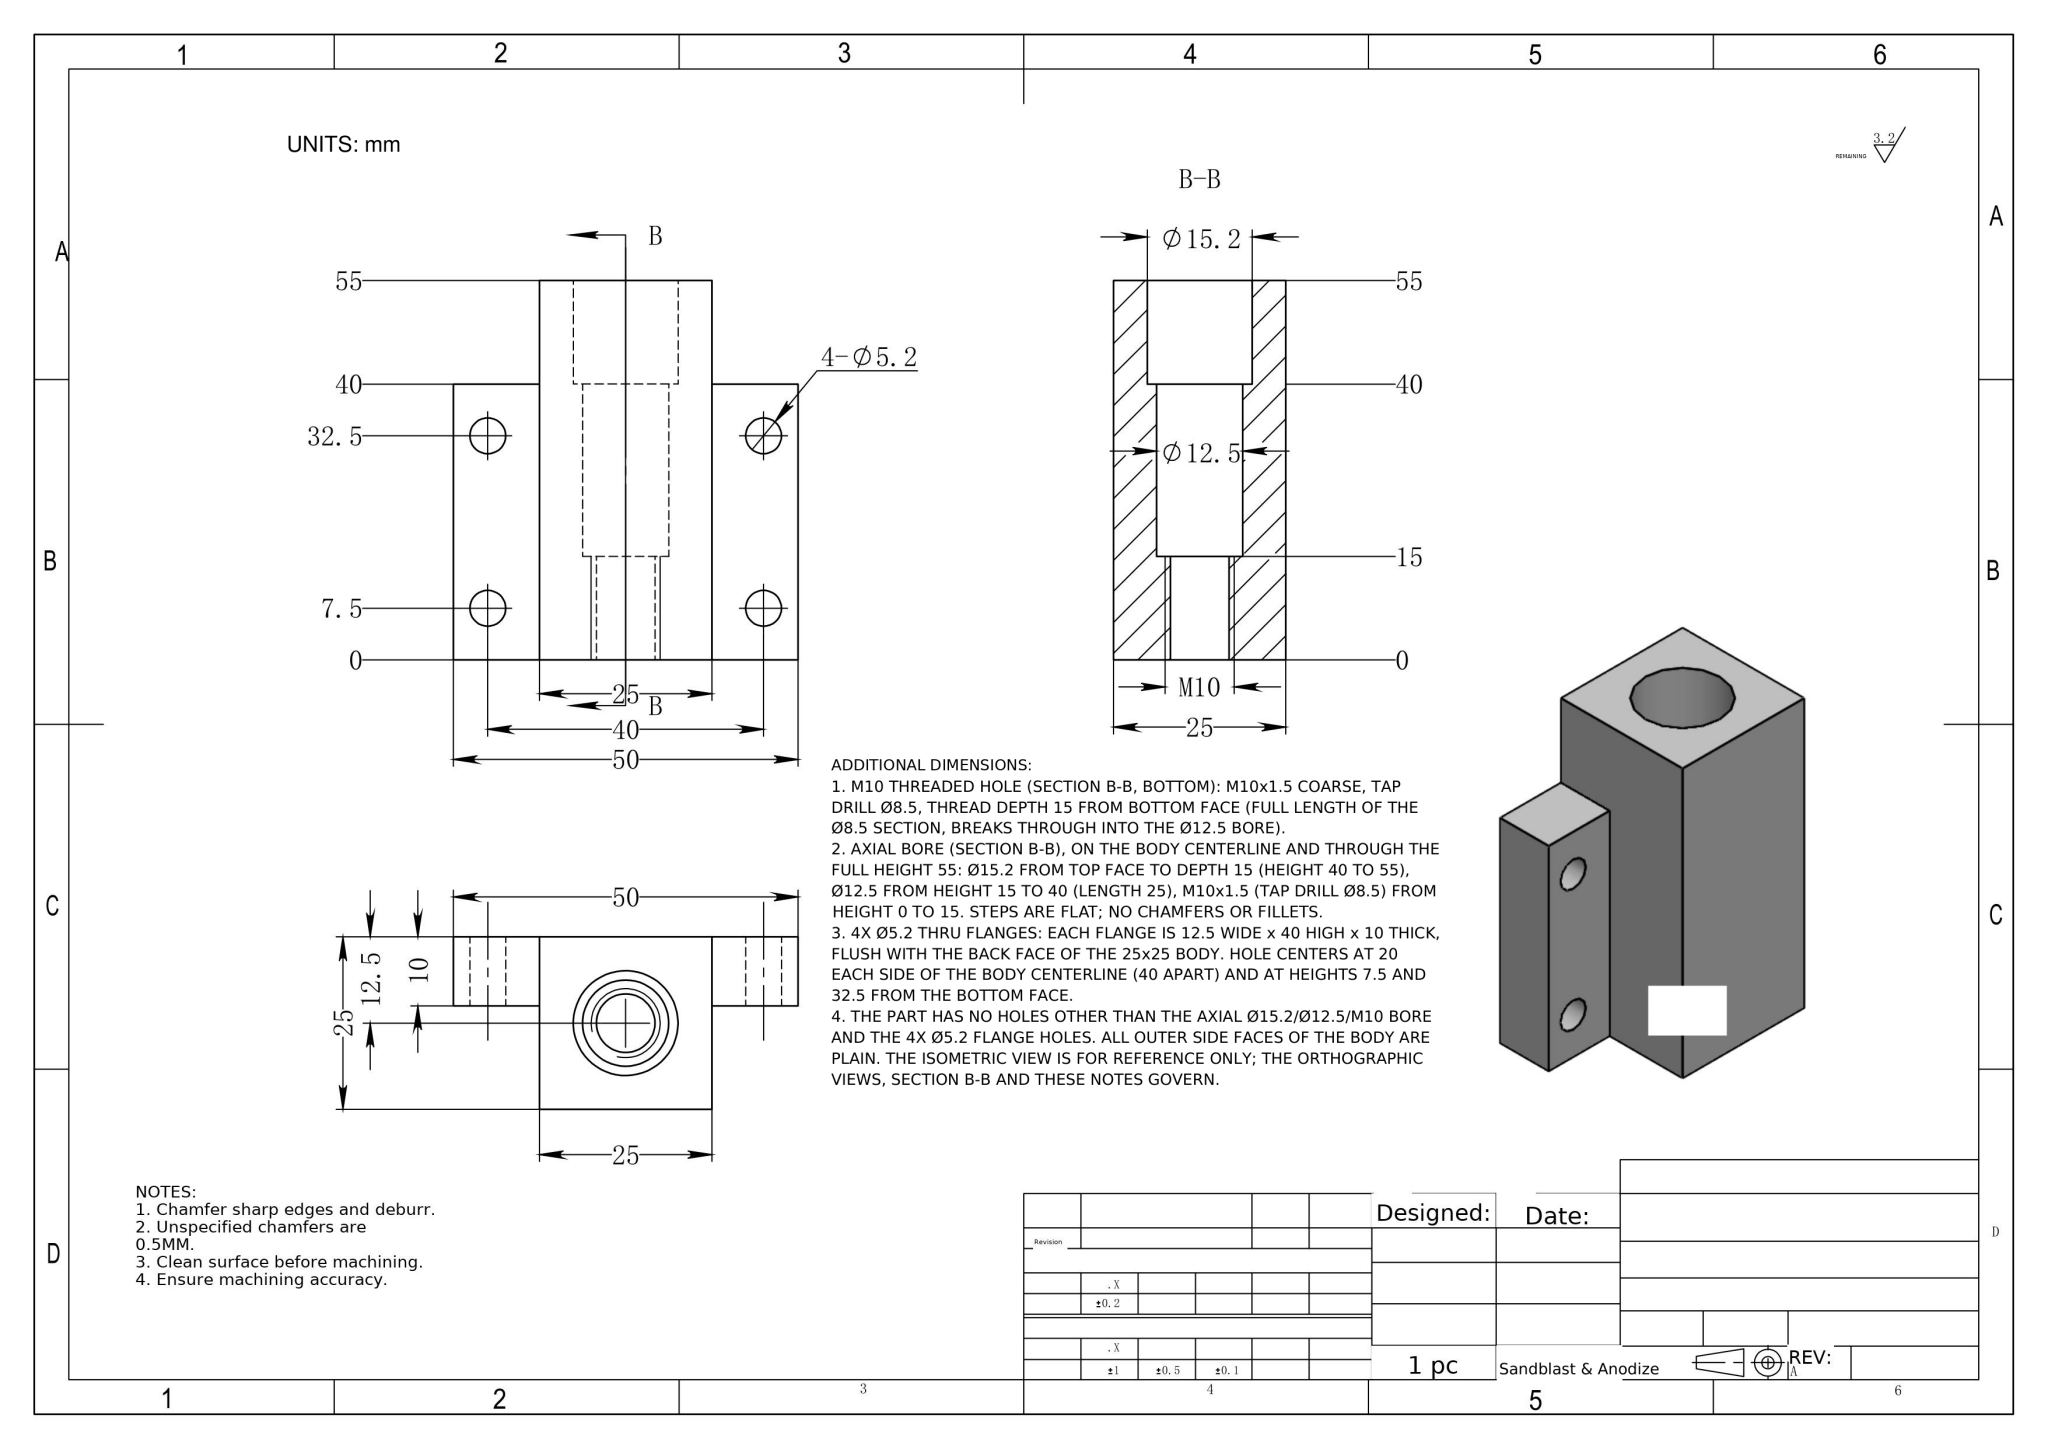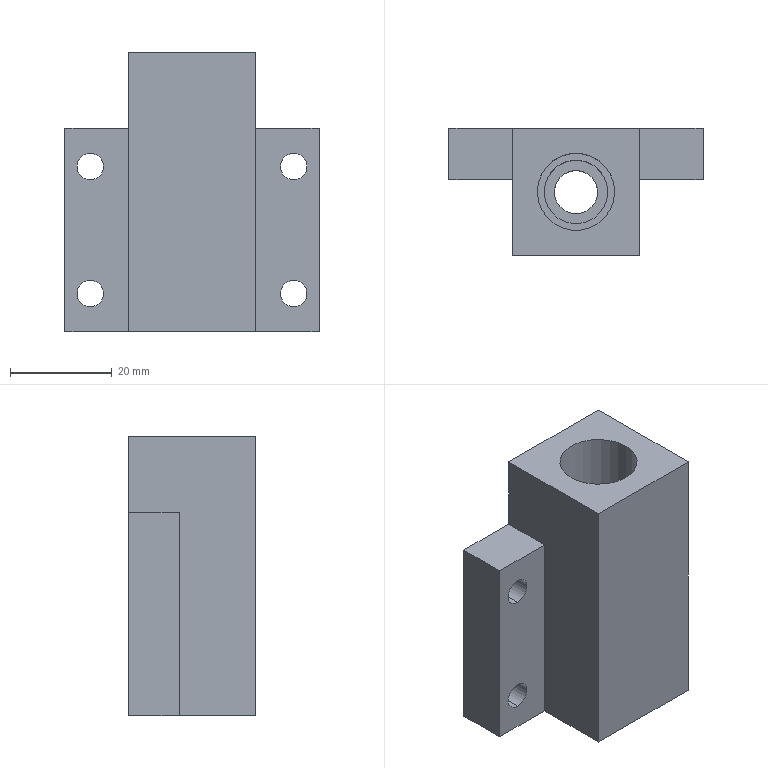Part | NX | mm | 1 solid | 28 faces | box 50 x 25 x 55 mm | volume 36885 mm3 | cylinder 14 | plane 14 | commonest cylinder face diameters 5.2 x8 8.5 x2 12.5 x2 15.2 x2
STEP:
#1=COLOUR_RGB('',1.,1.,1.);
#2=FILL_AREA_STYLE_COLOUR('',#1);
#3=FILL_AREA_STYLE('',(#2));
#4=SURFACE_STYLE_FILL_AREA(#3);
#5=SURFACE_SIDE_STYLE('',(#4));
#6=SURFACE_STYLE_USAGE(.BOTH.,#5);
#7=PRESENTATION_STYLE_ASSIGNMENT((#6));
#8=CARTESIAN_POINT('',(-4.25,0.,15.));
#9=VERTEX_POINT('',#8);
#10=CARTESIAN_POINT('',(4.25,0.,15.));
#11=VERTEX_POINT('',#10);
#12=CARTESIAN_POINT('',(0.,0.,15.));
#13=DIRECTION('',(0.,0.,1.));
#14=DIRECTION('',(1.,0.,0.));
#15=AXIS2_PLACEMENT_3D('',#12,#13,#14);
#16=CIRCLE('',#15,4.25);
#17=EDGE_CURVE('',#9,#11,#16,.T.);
#18=ORIENTED_EDGE('',*,*,#17,.T.);
#19=CARTESIAN_POINT('',(4.25,0.,0.));
#20=VERTEX_POINT('',#19);
#21=CARTESIAN_POINT('',(4.25,0.,0.));
#22=DIRECTION('',(0.,0.,-1.));
#23=VECTOR('',#22,1000.);
#24=LINE('',#21,#23);
#25=EDGE_CURVE('',#11,#20,#24,.T.);
#26=ORIENTED_EDGE('',*,*,#25,.T.);
#27=CARTESIAN_POINT('',(-4.25,0.,0.));
#28=VERTEX_POINT('',#27);
#29=CARTESIAN_POINT('',(0.,0.,0.));
#30=DIRECTION('',(0.,0.,-1.));
#31=DIRECTION('',(-1.,0.,0.));
#32=AXIS2_PLACEMENT_3D('',#29,#30,#31);
#33=CIRCLE('',#32,4.25);
#34=EDGE_CURVE('',#20,#28,#33,.T.);
#35=ORIENTED_EDGE('',*,*,#34,.T.);
#36=CARTESIAN_POINT('',(-4.25,0.,0.));
#37=DIRECTION('',(0.,0.,-1.));
#38=VECTOR('',#37,1000.);
#39=LINE('',#36,#38);
#40=EDGE_CURVE('',#9,#28,#39,.T.);
#41=ORIENTED_EDGE('',*,*,#40,.F.);
#42=EDGE_LOOP('',(#18,#26,#35,#41));
#43=FACE_OUTER_BOUND('',#42,.T.);
#44=CARTESIAN_POINT('',(0.,0.,0.));
#45=DIRECTION('',(0.,0.,-1.));
#46=DIRECTION('',(-1.,0.,0.));
#47=AXIS2_PLACEMENT_3D('',#44,#45,#46);
#48=CYLINDRICAL_SURFACE('',#47,4.25);
#49=ADVANCED_FACE('',(#43),#48,.F.);
#50=CARTESIAN_POINT('',(-6.25,0.,15.));
#51=VERTEX_POINT('',#50);
#52=CARTESIAN_POINT('',(6.25,0.,15.));
#53=VERTEX_POINT('',#52);
#54=CARTESIAN_POINT('',(0.,0.,15.));
#55=DIRECTION('',(0.,0.,1.));
#56=DIRECTION('',(1.,0.,0.));
#57=AXIS2_PLACEMENT_3D('',#54,#55,#56);
#58=CIRCLE('',#57,6.25);
#59=EDGE_CURVE('',#51,#53,#58,.T.);
#60=ORIENTED_EDGE('',*,*,#59,.F.);
#61=CARTESIAN_POINT('',(-6.25,0.,40.));
#62=VERTEX_POINT('',#61);
#63=CARTESIAN_POINT('',(-6.25,0.,15.));
#64=DIRECTION('',(0.,0.,1.));
#65=VECTOR('',#64,1000.);
#66=LINE('',#63,#65);
#67=EDGE_CURVE('',#51,#62,#66,.T.);
#68=ORIENTED_EDGE('',*,*,#67,.T.);
#69=CARTESIAN_POINT('',(6.25,0.,40.));
#70=VERTEX_POINT('',#69);
#71=CARTESIAN_POINT('',(0.,0.,40.));
#72=DIRECTION('',(0.,0.,1.));
#73=DIRECTION('',(1.,0.,0.));
#74=AXIS2_PLACEMENT_3D('',#71,#72,#73);
#75=CIRCLE('',#74,6.25);
#76=EDGE_CURVE('',#62,#70,#75,.T.);
#77=ORIENTED_EDGE('',*,*,#76,.T.);
#78=CARTESIAN_POINT('',(6.25,0.,15.));
#79=DIRECTION('',(0.,0.,1.));
#80=VECTOR('',#79,1000.);
#81=LINE('',#78,#80);
#82=EDGE_CURVE('',#53,#70,#81,.T.);
#83=ORIENTED_EDGE('',*,*,#82,.F.);
#84=EDGE_LOOP('',(#60,#68,#77,#83));
#85=FACE_OUTER_BOUND('',#84,.T.);
#86=CARTESIAN_POINT('',(0.,0.,15.));
#87=DIRECTION('',(0.,0.,1.));
#88=DIRECTION('',(1.,0.,0.));
#89=AXIS2_PLACEMENT_3D('',#86,#87,#88);
#90=CYLINDRICAL_SURFACE('',#89,6.25);
#91=ADVANCED_FACE('',(#85),#90,.F.);
#92=CARTESIAN_POINT('',(-7.6,0.,40.));
#93=VERTEX_POINT('',#92);
#94=CARTESIAN_POINT('',(7.6,0.,40.));
#95=VERTEX_POINT('',#94);
#96=CARTESIAN_POINT('',(0.,0.,40.));
#97=DIRECTION('',(0.,0.,1.));
#98=DIRECTION('',(1.,0.,0.));
#99=AXIS2_PLACEMENT_3D('',#96,#97,#98);
#100=CIRCLE('',#99,7.6);
#101=EDGE_CURVE('',#93,#95,#100,.T.);
#102=ORIENTED_EDGE('',*,*,#101,.F.);
#103=CARTESIAN_POINT('',(-7.6,0.,55.));
#104=VERTEX_POINT('',#103);
#105=CARTESIAN_POINT('',(-7.6,0.,40.));
#106=DIRECTION('',(0.,0.,1.));
#107=VECTOR('',#106,1000.);
#108=LINE('',#105,#107);
#109=EDGE_CURVE('',#93,#104,#108,.T.);
#110=ORIENTED_EDGE('',*,*,#109,.T.);
#111=CARTESIAN_POINT('',(7.6,0.,55.));
#112=VERTEX_POINT('',#111);
#113=CARTESIAN_POINT('',(0.,0.,55.));
#114=DIRECTION('',(0.,0.,1.));
#115=DIRECTION('',(1.,0.,0.));
#116=AXIS2_PLACEMENT_3D('',#113,#114,#115);
#117=CIRCLE('',#116,7.6);
#118=EDGE_CURVE('',#104,#112,#117,.T.);
#119=ORIENTED_EDGE('',*,*,#118,.T.);
#120=CARTESIAN_POINT('',(7.6,0.,40.));
#121=DIRECTION('',(0.,0.,1.));
#122=VECTOR('',#121,1000.);
#123=LINE('',#120,#122);
#124=EDGE_CURVE('',#95,#112,#123,.T.);
#125=ORIENTED_EDGE('',*,*,#124,.F.);
#126=EDGE_LOOP('',(#102,#110,#119,#125));
#127=FACE_OUTER_BOUND('',#126,.T.);
#128=CARTESIAN_POINT('',(0.,0.,40.));
#129=DIRECTION('',(0.,0.,1.));
#130=DIRECTION('',(1.,0.,0.));
#131=AXIS2_PLACEMENT_3D('',#128,#129,#130);
#132=CYLINDRICAL_SURFACE('',#131,7.6);
#133=ADVANCED_FACE('',(#127),#132,.F.);
#134=CARTESIAN_POINT('',(-20.,12.5,35.1));
#135=VERTEX_POINT('',#134);
#136=CARTESIAN_POINT('',(-20.,12.5,29.9));
#137=VERTEX_POINT('',#136);
#138=CARTESIAN_POINT('',(-20.,12.5,32.5));
#139=DIRECTION('',(0.,-1.,0.));
#140=DIRECTION('',(0.,0.,-1.));
#141=AXIS2_PLACEMENT_3D('',#138,#139,#140);
#142=CIRCLE('',#141,2.6);
#143=EDGE_CURVE('',#135,#137,#142,.T.);
#144=ORIENTED_EDGE('',*,*,#143,.F.);
#145=CARTESIAN_POINT('',(-20.,2.5,35.1));
#146=VERTEX_POINT('',#145);
#147=CARTESIAN_POINT('',(-20.,-12.5,35.1));
#148=DIRECTION('',(0.,-1.,0.));
#149=VECTOR('',#148,1000.);
#150=LINE('',#147,#149);
#151=EDGE_CURVE('',#135,#146,#150,.T.);
#152=ORIENTED_EDGE('',*,*,#151,.T.);
#153=CARTESIAN_POINT('',(-20.,2.5,29.9));
#154=VERTEX_POINT('',#153);
#155=CARTESIAN_POINT('',(-20.,2.5,32.5));
#156=DIRECTION('',(0.,1.,0.));
#157=DIRECTION('',(0.,0.,-1.));
#158=AXIS2_PLACEMENT_3D('',#155,#156,#157);
#159=CIRCLE('',#158,2.6);
#160=EDGE_CURVE('',#154,#146,#159,.T.);
#161=ORIENTED_EDGE('',*,*,#160,.F.);
#162=CARTESIAN_POINT('',(-20.,-12.5,29.9));
#163=DIRECTION('',(0.,-1.,0.));
#164=VECTOR('',#163,1000.);
#165=LINE('',#162,#164);
#166=EDGE_CURVE('',#137,#154,#165,.T.);
#167=ORIENTED_EDGE('',*,*,#166,.F.);
#168=EDGE_LOOP('',(#144,#152,#161,#167));
#169=FACE_OUTER_BOUND('',#168,.T.);
#170=CARTESIAN_POINT('',(-20.,-12.5,32.5));
#171=DIRECTION('',(0.,-1.,0.));
#172=DIRECTION('',(0.,0.,-1.));
#173=AXIS2_PLACEMENT_3D('',#170,#171,#172);
#174=CYLINDRICAL_SURFACE('',#173,2.6);
#175=ADVANCED_FACE('',(#169),#174,.F.);
#176=CARTESIAN_POINT('',(-20.,12.5,10.1));
#177=VERTEX_POINT('',#176);
#178=CARTESIAN_POINT('',(-20.,12.5,4.9));
#179=VERTEX_POINT('',#178);
#180=CARTESIAN_POINT('',(-20.,12.5,7.5));
#181=DIRECTION('',(0.,-1.,0.));
#182=DIRECTION('',(0.,0.,-1.));
#183=AXIS2_PLACEMENT_3D('',#180,#181,#182);
#184=CIRCLE('',#183,2.6);
#185=EDGE_CURVE('',#177,#179,#184,.T.);
#186=ORIENTED_EDGE('',*,*,#185,.F.);
#187=CARTESIAN_POINT('',(-20.,2.5,10.1));
#188=VERTEX_POINT('',#187);
#189=CARTESIAN_POINT('',(-20.,-12.5,10.1));
#190=DIRECTION('',(0.,-1.,0.));
#191=VECTOR('',#190,1000.);
#192=LINE('',#189,#191);
#193=EDGE_CURVE('',#177,#188,#192,.T.);
#194=ORIENTED_EDGE('',*,*,#193,.T.);
#195=CARTESIAN_POINT('',(-20.,2.5,4.9));
#196=VERTEX_POINT('',#195);
#197=CARTESIAN_POINT('',(-20.,2.5,7.5));
#198=DIRECTION('',(0.,1.,0.));
#199=DIRECTION('',(0.,0.,-1.));
#200=AXIS2_PLACEMENT_3D('',#197,#198,#199);
#201=CIRCLE('',#200,2.6);
#202=EDGE_CURVE('',#196,#188,#201,.T.);
#203=ORIENTED_EDGE('',*,*,#202,.F.);
#204=CARTESIAN_POINT('',(-20.,-12.5,4.9));
#205=DIRECTION('',(0.,-1.,0.));
#206=VECTOR('',#205,1000.);
#207=LINE('',#204,#206);
#208=EDGE_CURVE('',#179,#196,#207,.T.);
#209=ORIENTED_EDGE('',*,*,#208,.F.);
#210=EDGE_LOOP('',(#186,#194,#203,#209));
#211=FACE_OUTER_BOUND('',#210,.T.);
#212=CARTESIAN_POINT('',(-20.,-12.5,7.5));
#213=DIRECTION('',(0.,-1.,0.));
#214=DIRECTION('',(0.,0.,-1.));
#215=AXIS2_PLACEMENT_3D('',#212,#213,#214);
#216=CYLINDRICAL_SURFACE('',#215,2.6);
#217=ADVANCED_FACE('',(#211),#216,.F.);
#218=CARTESIAN_POINT('',(20.,12.5,35.1));
#219=VERTEX_POINT('',#218);
#220=CARTESIAN_POINT('',(20.,12.5,29.9));
#221=VERTEX_POINT('',#220);
#222=CARTESIAN_POINT('',(20.,12.5,32.5));
#223=DIRECTION('',(0.,-1.,0.));
#224=DIRECTION('',(0.,0.,-1.));
#225=AXIS2_PLACEMENT_3D('',#222,#223,#224);
#226=CIRCLE('',#225,2.6);
#227=EDGE_CURVE('',#219,#221,#226,.T.);
#228=ORIENTED_EDGE('',*,*,#227,.F.);
#229=CARTESIAN_POINT('',(20.,2.5,35.1));
#230=VERTEX_POINT('',#229);
#231=CARTESIAN_POINT('',(20.,-12.5,35.1));
#232=DIRECTION('',(0.,-1.,0.));
#233=VECTOR('',#232,1000.);
#234=LINE('',#231,#233);
#235=EDGE_CURVE('',#219,#230,#234,.T.);
#236=ORIENTED_EDGE('',*,*,#235,.T.);
#237=CARTESIAN_POINT('',(20.,2.5,29.9));
#238=VERTEX_POINT('',#237);
#239=CARTESIAN_POINT('',(20.,2.5,32.5));
#240=DIRECTION('',(0.,1.,0.));
#241=DIRECTION('',(0.,0.,-1.));
#242=AXIS2_PLACEMENT_3D('',#239,#240,#241);
#243=CIRCLE('',#242,2.6);
#244=EDGE_CURVE('',#238,#230,#243,.T.);
#245=ORIENTED_EDGE('',*,*,#244,.F.);
#246=CARTESIAN_POINT('',(20.,-12.5,29.9));
#247=DIRECTION('',(0.,-1.,0.));
#248=VECTOR('',#247,1000.);
#249=LINE('',#246,#248);
#250=EDGE_CURVE('',#221,#238,#249,.T.);
#251=ORIENTED_EDGE('',*,*,#250,.F.);
#252=EDGE_LOOP('',(#228,#236,#245,#251));
#253=FACE_OUTER_BOUND('',#252,.T.);
#254=CARTESIAN_POINT('',(20.,-12.5,32.5));
#255=DIRECTION('',(0.,-1.,0.));
#256=DIRECTION('',(0.,0.,-1.));
#257=AXIS2_PLACEMENT_3D('',#254,#255,#256);
#258=CYLINDRICAL_SURFACE('',#257,2.6);
#259=ADVANCED_FACE('',(#253),#258,.F.);
#260=CARTESIAN_POINT('',(20.,12.5,10.1));
#261=VERTEX_POINT('',#260);
#262=CARTESIAN_POINT('',(20.,12.5,4.9));
#263=VERTEX_POINT('',#262);
#264=CARTESIAN_POINT('',(20.,12.5,7.5));
#265=DIRECTION('',(0.,-1.,0.));
#266=DIRECTION('',(0.,0.,-1.));
#267=AXIS2_PLACEMENT_3D('',#264,#265,#266);
#268=CIRCLE('',#267,2.6);
#269=EDGE_CURVE('',#261,#263,#268,.T.);
#270=ORIENTED_EDGE('',*,*,#269,.F.);
#271=CARTESIAN_POINT('',(20.,2.5,10.1));
#272=VERTEX_POINT('',#271);
#273=CARTESIAN_POINT('',(20.,-12.5,10.1));
#274=DIRECTION('',(0.,-1.,0.));
#275=VECTOR('',#274,1000.);
#276=LINE('',#273,#275);
#277=EDGE_CURVE('',#261,#272,#276,.T.);
#278=ORIENTED_EDGE('',*,*,#277,.T.);
#279=CARTESIAN_POINT('',(20.,2.5,4.9));
#280=VERTEX_POINT('',#279);
#281=CARTESIAN_POINT('',(20.,2.5,7.5));
#282=DIRECTION('',(0.,1.,0.));
#283=DIRECTION('',(0.,0.,-1.));
#284=AXIS2_PLACEMENT_3D('',#281,#282,#283);
#285=CIRCLE('',#284,2.6);
#286=EDGE_CURVE('',#280,#272,#285,.T.);
#287=ORIENTED_EDGE('',*,*,#286,.F.);
#288=CARTESIAN_POINT('',(20.,-12.5,4.9));
#289=DIRECTION('',(0.,-1.,0.));
#290=VECTOR('',#289,1000.);
#291=LINE('',#288,#290);
#292=EDGE_CURVE('',#263,#280,#291,.T.);
#293=ORIENTED_EDGE('',*,*,#292,.F.);
#294=EDGE_LOOP('',(#270,#278,#287,#293));
#295=FACE_OUTER_BOUND('',#294,.T.);
#296=CARTESIAN_POINT('',(20.,-12.5,7.5));
#297=DIRECTION('',(0.,-1.,0.));
#298=DIRECTION('',(0.,0.,-1.));
#299=AXIS2_PLACEMENT_3D('',#296,#297,#298);
#300=CYLINDRICAL_SURFACE('',#299,2.6);
#301=ADVANCED_FACE('',(#295),#300,.F.);
#302=CARTESIAN_POINT('',(25.,2.5,0.));
#303=VERTEX_POINT('',#302);
#304=CARTESIAN_POINT('',(25.,2.5,40.));
#305=VERTEX_POINT('',#304);
#306=CARTESIAN_POINT('',(25.,2.5,55.));
#307=DIRECTION('',(0.,0.,1.));
#308=VECTOR('',#307,1000.);
#309=LINE('',#306,#308);
#310=EDGE_CURVE('',#303,#305,#309,.T.);
#311=ORIENTED_EDGE('',*,*,#310,.F.);
#312=CARTESIAN_POINT('',(25.,12.5,0.));
#313=VERTEX_POINT('',#312);
#314=CARTESIAN_POINT('',(25.,12.5,0.));
#315=DIRECTION('',(0.,1.,0.));
#316=VECTOR('',#315,1000.);
#317=LINE('',#314,#316);
#318=EDGE_CURVE('',#303,#313,#317,.T.);
#319=ORIENTED_EDGE('',*,*,#318,.T.);
#320=CARTESIAN_POINT('',(25.,12.5,40.));
#321=VERTEX_POINT('',#320);
#322=CARTESIAN_POINT('',(25.,12.5,55.));
#323=DIRECTION('',(0.,0.,-1.));
#324=VECTOR('',#323,1000.);
#325=LINE('',#322,#324);
#326=EDGE_CURVE('',#321,#313,#325,.T.);
#327=ORIENTED_EDGE('',*,*,#326,.F.);
#328=CARTESIAN_POINT('',(25.,12.5,40.));
#329=DIRECTION('',(0.,1.,0.));
#330=VECTOR('',#329,1000.);
#331=LINE('',#328,#330);
#332=EDGE_CURVE('',#305,#321,#331,.T.);
#333=ORIENTED_EDGE('',*,*,#332,.F.);
#334=EDGE_LOOP('',(#311,#319,#327,#333));
#335=FACE_OUTER_BOUND('',#334,.T.);
#336=CARTESIAN_POINT('',(25.,12.5,55.));
#337=DIRECTION('',(-1.,0.,0.));
#338=DIRECTION('',(0.,0.,1.));
#339=AXIS2_PLACEMENT_3D('',#336,#337,#338);
#340=PLANE('',#339);
#341=ADVANCED_FACE('',(#335),#340,.F.);
#342=CARTESIAN_POINT('',(-25.,2.5,40.));
#343=VERTEX_POINT('',#342);
#344=CARTESIAN_POINT('',(-25.,2.5,0.));
#345=VERTEX_POINT('',#344);
#346=CARTESIAN_POINT('',(-25.,2.5,55.));
#347=DIRECTION('',(0.,0.,-1.));
#348=VECTOR('',#347,1000.);
#349=LINE('',#346,#348);
#350=EDGE_CURVE('',#343,#345,#349,.T.);
#351=ORIENTED_EDGE('',*,*,#350,.F.);
#352=CARTESIAN_POINT('',(-25.,12.5,40.));
#353=VERTEX_POINT('',#352);
#354=CARTESIAN_POINT('',(-25.,12.5,40.));
#355=DIRECTION('',(0.,-1.,0.));
#356=VECTOR('',#355,1000.);
#357=LINE('',#354,#356);
#358=EDGE_CURVE('',#353,#343,#357,.T.);
#359=ORIENTED_EDGE('',*,*,#358,.F.);
#360=CARTESIAN_POINT('',(-25.,12.5,0.));
#361=VERTEX_POINT('',#360);
#362=CARTESIAN_POINT('',(-25.,12.5,55.));
#363=DIRECTION('',(0.,0.,-1.));
#364=VECTOR('',#363,1000.);
#365=LINE('',#362,#364);
#366=EDGE_CURVE('',#353,#361,#365,.T.);
#367=ORIENTED_EDGE('',*,*,#366,.T.);
#368=CARTESIAN_POINT('',(-25.,12.5,0.));
#369=DIRECTION('',(0.,-1.,0.));
#370=VECTOR('',#369,1000.);
#371=LINE('',#368,#370);
#372=EDGE_CURVE('',#361,#345,#371,.T.);
#373=ORIENTED_EDGE('',*,*,#372,.T.);
#374=EDGE_LOOP('',(#351,#359,#367,#373));
#375=FACE_OUTER_BOUND('',#374,.T.);
#376=CARTESIAN_POINT('',(-25.,12.5,55.));
#377=DIRECTION('',(1.,0.,0.));
#378=DIRECTION('',(-0.,1.,0.));
#379=AXIS2_PLACEMENT_3D('',#376,#377,#378);
#380=PLANE('',#379);
#381=ADVANCED_FACE('',(#375),#380,.F.);
#382=CARTESIAN_POINT('',(-12.5,-12.5,0.));
#383=VERTEX_POINT('',#382);
#384=CARTESIAN_POINT('',(12.5,-12.5,0.));
#385=VERTEX_POINT('',#384);
#386=CARTESIAN_POINT('',(-25.,-12.5,0.));
#387=DIRECTION('',(1.,0.,0.));
#388=VECTOR('',#387,1000.);
#389=LINE('',#386,#388);
#390=EDGE_CURVE('',#383,#385,#389,.T.);
#391=ORIENTED_EDGE('',*,*,#390,.T.);
#392=CARTESIAN_POINT('',(12.5,-12.5,55.));
#393=VERTEX_POINT('',#392);
#394=CARTESIAN_POINT('',(12.5,-12.5,40.));
#395=DIRECTION('',(0.,0.,1.));
#396=VECTOR('',#395,1000.);
#397=LINE('',#394,#396);
#398=EDGE_CURVE('',#385,#393,#397,.T.);
#399=ORIENTED_EDGE('',*,*,#398,.T.);
#400=CARTESIAN_POINT('',(-12.5,-12.5,55.));
#401=VERTEX_POINT('',#400);
#402=CARTESIAN_POINT('',(-25.,-12.5,55.));
#403=DIRECTION('',(1.,0.,0.));
#404=VECTOR('',#403,1000.);
#405=LINE('',#402,#404);
#406=EDGE_CURVE('',#401,#393,#405,.T.);
#407=ORIENTED_EDGE('',*,*,#406,.F.);
#408=CARTESIAN_POINT('',(-12.5,-12.5,40.));
#409=DIRECTION('',(0.,0.,1.));
#410=VECTOR('',#409,1000.);
#411=LINE('',#408,#410);
#412=EDGE_CURVE('',#383,#401,#411,.T.);
#413=ORIENTED_EDGE('',*,*,#412,.F.);
#414=EDGE_LOOP('',(#391,#399,#407,#413));
#415=FACE_OUTER_BOUND('',#414,.T.);
#416=CARTESIAN_POINT('',(-25.,-12.5,55.));
#417=DIRECTION('',(0.,1.,0.));
#418=DIRECTION('',(0.,0.,1.));
#419=AXIS2_PLACEMENT_3D('',#416,#417,#418);
#420=PLANE('',#419);
#421=ADVANCED_FACE('',(#415),#420,.F.);
#422=CARTESIAN_POINT('',(0.,0.,0.));
#423=DIRECTION('',(0.,0.,-1.));
#424=DIRECTION('',(-1.,0.,0.));
#425=AXIS2_PLACEMENT_3D('',#422,#423,#424);
#426=CIRCLE('',#425,4.25);
#427=EDGE_CURVE('',#28,#20,#426,.T.);
#428=ORIENTED_EDGE('',*,*,#427,.F.);
#429=ORIENTED_EDGE('',*,*,#34,.F.);
#430=EDGE_LOOP('',(#428,#429));
#431=FACE_BOUND('',#430,.T.);
#432=CARTESIAN_POINT('',(12.5,2.5,0.));
#433=VERTEX_POINT('',#432);
#434=CARTESIAN_POINT('',(0.,2.5,0.));
#435=DIRECTION('',(1.,0.,0.));
#436=VECTOR('',#435,1000.);
#437=LINE('',#434,#436);
#438=EDGE_CURVE('',#433,#303,#437,.T.);
#439=ORIENTED_EDGE('',*,*,#438,.F.);
#440=CARTESIAN_POINT('',(12.5,0.,0.));
#441=DIRECTION('',(0.,1.,0.));
#442=VECTOR('',#441,1000.);
#443=LINE('',#440,#442);
#444=EDGE_CURVE('',#385,#433,#443,.T.);
#445=ORIENTED_EDGE('',*,*,#444,.F.);
#446=ORIENTED_EDGE('',*,*,#390,.F.);
#447=CARTESIAN_POINT('',(-12.5,2.5,0.));
#448=VERTEX_POINT('',#447);
#449=CARTESIAN_POINT('',(-12.5,0.,0.));
#450=DIRECTION('',(0.,-1.,0.));
#451=VECTOR('',#450,1000.);
#452=LINE('',#449,#451);
#453=EDGE_CURVE('',#448,#383,#452,.T.);
#454=ORIENTED_EDGE('',*,*,#453,.F.);
#455=CARTESIAN_POINT('',(0.,2.5,0.));
#456=DIRECTION('',(1.,0.,0.));
#457=VECTOR('',#456,1000.);
#458=LINE('',#455,#457);
#459=EDGE_CURVE('',#345,#448,#458,.T.);
#460=ORIENTED_EDGE('',*,*,#459,.F.);
#461=ORIENTED_EDGE('',*,*,#372,.F.);
#462=CARTESIAN_POINT('',(-25.,12.5,0.));
#463=DIRECTION('',(-1.,0.,0.));
#464=VECTOR('',#463,1000.);
#465=LINE('',#462,#464);
#466=EDGE_CURVE('',#313,#361,#465,.T.);
#467=ORIENTED_EDGE('',*,*,#466,.F.);
#468=ORIENTED_EDGE('',*,*,#318,.F.);
#469=EDGE_LOOP('',(#439,#445,#446,#454,#460,#461,#467,#468));
#470=FACE_OUTER_BOUND('',#469,.T.);
#471=CARTESIAN_POINT('',(0.,0.,0.));
#472=DIRECTION('',(0.,0.,1.));
#473=DIRECTION('',(1.,0.,0.));
#474=AXIS2_PLACEMENT_3D('',#471,#472,#473);
#475=PLANE('',#474);
#476=ADVANCED_FACE('',(#431,#470),#475,.F.);
#477=ORIENTED_EDGE('',*,*,#358,.T.);
#478=CARTESIAN_POINT('',(-12.5,2.5,40.));
#479=VERTEX_POINT('',#478);
#480=CARTESIAN_POINT('',(0.,2.5,40.));
#481=DIRECTION('',(1.,0.,0.));
#482=VECTOR('',#481,1000.);
#483=LINE('',#480,#482);
#484=EDGE_CURVE('',#343,#479,#483,.T.);
#485=ORIENTED_EDGE('',*,*,#484,.T.);
#486=CARTESIAN_POINT('',(-12.5,12.5,40.));
#487=VERTEX_POINT('',#486);
#488=CARTESIAN_POINT('',(-12.5,12.5,40.));
#489=DIRECTION('',(0.,-1.,0.));
#490=VECTOR('',#489,1000.);
#491=LINE('',#488,#490);
#492=EDGE_CURVE('',#487,#479,#491,.T.);
#493=ORIENTED_EDGE('',*,*,#492,.F.);
#494=CARTESIAN_POINT('',(-25.,12.5,40.));
#495=DIRECTION('',(-1.,0.,0.));
#496=VECTOR('',#495,1000.);
#497=LINE('',#494,#496);
#498=EDGE_CURVE('',#487,#353,#497,.T.);
#499=ORIENTED_EDGE('',*,*,#498,.T.);
#500=EDGE_LOOP('',(#477,#485,#493,#499));
#501=FACE_OUTER_BOUND('',#500,.T.);
#502=CARTESIAN_POINT('',(0.,0.,40.));
#503=DIRECTION('',(0.,0.,1.));
#504=DIRECTION('',(1.,0.,0.));
#505=AXIS2_PLACEMENT_3D('',#502,#503,#504);
#506=PLANE('',#505);
#507=ADVANCED_FACE('',(#501),#506,.T.);
#508=CARTESIAN_POINT('',(12.5,2.5,40.));
#509=VERTEX_POINT('',#508);
#510=CARTESIAN_POINT('',(12.5,12.5,40.));
#511=VERTEX_POINT('',#510);
#512=CARTESIAN_POINT('',(12.5,12.5,40.));
#513=DIRECTION('',(0.,1.,0.));
#514=VECTOR('',#513,1000.);
#515=LINE('',#512,#514);
#516=EDGE_CURVE('',#509,#511,#515,.T.);
#517=ORIENTED_EDGE('',*,*,#516,.F.);
#518=CARTESIAN_POINT('',(0.,2.5,40.));
#519=DIRECTION('',(1.,0.,0.));
#520=VECTOR('',#519,1000.);
#521=LINE('',#518,#520);
#522=EDGE_CURVE('',#509,#305,#521,.T.);
#523=ORIENTED_EDGE('',*,*,#522,.T.);
#524=ORIENTED_EDGE('',*,*,#332,.T.);
#525=CARTESIAN_POINT('',(-25.,12.5,40.));
#526=DIRECTION('',(-1.,0.,0.));
#527=VECTOR('',#526,1000.);
#528=LINE('',#525,#527);
#529=EDGE_CURVE('',#321,#511,#528,.T.);
#530=ORIENTED_EDGE('',*,*,#529,.T.);
#531=EDGE_LOOP('',(#517,#523,#524,#530));
#532=FACE_OUTER_BOUND('',#531,.T.);
#533=CARTESIAN_POINT('',(0.,0.,40.));
#534=DIRECTION('',(0.,0.,1.));
#535=DIRECTION('',(1.,0.,0.));
#536=AXIS2_PLACEMENT_3D('',#533,#534,#535);
#537=PLANE('',#536);
#538=ADVANCED_FACE('',(#532),#537,.T.);
#539=ORIENTED_EDGE('',*,*,#277,.F.);
#540=CARTESIAN_POINT('',(20.,12.5,7.5));
#541=DIRECTION('',(0.,-1.,0.));
#542=DIRECTION('',(0.,0.,-1.));
#543=AXIS2_PLACEMENT_3D('',#540,#541,#542);
#544=CIRCLE('',#543,2.6);
#545=EDGE_CURVE('',#263,#261,#544,.T.);
#546=ORIENTED_EDGE('',*,*,#545,.F.);
#547=ORIENTED_EDGE('',*,*,#292,.T.);
#548=CARTESIAN_POINT('',(20.,2.5,7.5));
#549=DIRECTION('',(0.,1.,0.));
#550=DIRECTION('',(0.,0.,-1.));
#551=AXIS2_PLACEMENT_3D('',#548,#549,#550);
#552=CIRCLE('',#551,2.6);
#553=EDGE_CURVE('',#272,#280,#552,.T.);
#554=ORIENTED_EDGE('',*,*,#553,.F.);
#555=EDGE_LOOP('',(#539,#546,#547,#554));
#556=FACE_OUTER_BOUND('',#555,.T.);
#557=CARTESIAN_POINT('',(20.,-12.5,7.5));
#558=DIRECTION('',(0.,-1.,0.));
#559=DIRECTION('',(0.,0.,-1.));
#560=AXIS2_PLACEMENT_3D('',#557,#558,#559);
#561=CYLINDRICAL_SURFACE('',#560,2.6);
#562=ADVANCED_FACE('',(#556),#561,.F.);
#563=ORIENTED_EDGE('',*,*,#235,.F.);
#564=CARTESIAN_POINT('',(20.,12.5,32.5));
#565=DIRECTION('',(0.,-1.,0.));
#566=DIRECTION('',(0.,0.,-1.));
#567=AXIS2_PLACEMENT_3D('',#564,#565,#566);
#568=CIRCLE('',#567,2.6);
#569=EDGE_CURVE('',#221,#219,#568,.T.);
#570=ORIENTED_EDGE('',*,*,#569,.F.);
#571=ORIENTED_EDGE('',*,*,#250,.T.);
#572=CARTESIAN_POINT('',(20.,2.5,32.5));
#573=DIRECTION('',(0.,1.,0.));
#574=DIRECTION('',(0.,0.,-1.));
#575=AXIS2_PLACEMENT_3D('',#572,#573,#574);
#576=CIRCLE('',#575,2.6);
#577=EDGE_CURVE('',#230,#238,#576,.T.);
#578=ORIENTED_EDGE('',*,*,#577,.F.);
#579=EDGE_LOOP('',(#563,#570,#571,#578));
#580=FACE_OUTER_BOUND('',#579,.T.);
#581=CARTESIAN_POINT('',(20.,-12.5,32.5));
#582=DIRECTION('',(0.,-1.,0.));
#583=DIRECTION('',(0.,0.,-1.));
#584=AXIS2_PLACEMENT_3D('',#581,#582,#583);
#585=CYLINDRICAL_SURFACE('',#584,2.6);
#586=ADVANCED_FACE('',(#580),#585,.F.);
#587=ORIENTED_EDGE('',*,*,#193,.F.);
#588=CARTESIAN_POINT('',(-20.,12.5,7.5));
#589=DIRECTION('',(0.,-1.,0.));
#590=DIRECTION('',(0.,0.,-1.));
#591=AXIS2_PLACEMENT_3D('',#588,#589,#590);
#592=CIRCLE('',#591,2.6);
#593=EDGE_CURVE('',#179,#177,#592,.T.);
#594=ORIENTED_EDGE('',*,*,#593,.F.);
#595=ORIENTED_EDGE('',*,*,#208,.T.);
#596=CARTESIAN_POINT('',(-20.,2.5,7.5));
#597=DIRECTION('',(0.,1.,0.));
#598=DIRECTION('',(0.,0.,-1.));
#599=AXIS2_PLACEMENT_3D('',#596,#597,#598);
#600=CIRCLE('',#599,2.6);
#601=EDGE_CURVE('',#188,#196,#600,.T.);
#602=ORIENTED_EDGE('',*,*,#601,.F.);
#603=EDGE_LOOP('',(#587,#594,#595,#602));
#604=FACE_OUTER_BOUND('',#603,.T.);
#605=CARTESIAN_POINT('',(-20.,-12.5,7.5));
#606=DIRECTION('',(0.,-1.,0.));
#607=DIRECTION('',(0.,0.,-1.));
#608=AXIS2_PLACEMENT_3D('',#605,#606,#607);
#609=CYLINDRICAL_SURFACE('',#608,2.6);
#610=ADVANCED_FACE('',(#604),#609,.F.);
#611=ORIENTED_EDGE('',*,*,#151,.F.);
#612=CARTESIAN_POINT('',(-20.,12.5,32.5));
#613=DIRECTION('',(0.,-1.,0.));
#614=DIRECTION('',(0.,0.,-1.));
#615=AXIS2_PLACEMENT_3D('',#612,#613,#614);
#616=CIRCLE('',#615,2.6);
#617=EDGE_CURVE('',#137,#135,#616,.T.);
#618=ORIENTED_EDGE('',*,*,#617,.F.);
#619=ORIENTED_EDGE('',*,*,#166,.T.);
#620=CARTESIAN_POINT('',(-20.,2.5,32.5));
#621=DIRECTION('',(0.,1.,0.));
#622=DIRECTION('',(0.,0.,-1.));
#623=AXIS2_PLACEMENT_3D('',#620,#621,#622);
#624=CIRCLE('',#623,2.6);
#625=EDGE_CURVE('',#146,#154,#624,.T.);
#626=ORIENTED_EDGE('',*,*,#625,.F.);
#627=EDGE_LOOP('',(#611,#618,#619,#626));
#628=FACE_OUTER_BOUND('',#627,.T.);
#629=CARTESIAN_POINT('',(-20.,-12.5,32.5));
#630=DIRECTION('',(0.,-1.,0.));
#631=DIRECTION('',(0.,0.,-1.));
#632=AXIS2_PLACEMENT_3D('',#629,#630,#631);
#633=CYLINDRICAL_SURFACE('',#632,2.6);
#634=ADVANCED_FACE('',(#628),#633,.F.);
#635=ORIENTED_EDGE('',*,*,#617,.T.);
#636=ORIENTED_EDGE('',*,*,#143,.T.);
#637=EDGE_LOOP('',(#635,#636));
#638=FACE_BOUND('',#637,.T.);
#639=ORIENTED_EDGE('',*,*,#593,.T.);
#640=ORIENTED_EDGE('',*,*,#185,.T.);
#641=EDGE_LOOP('',(#639,#640));
#642=FACE_BOUND('',#641,.T.);
#643=ORIENTED_EDGE('',*,*,#569,.T.);
#644=ORIENTED_EDGE('',*,*,#227,.T.);
#645=EDGE_LOOP('',(#643,#644));
#646=FACE_BOUND('',#645,.T.);
#647=ORIENTED_EDGE('',*,*,#545,.T.);
#648=ORIENTED_EDGE('',*,*,#269,.T.);
#649=EDGE_LOOP('',(#647,#648));
#650=FACE_BOUND('',#649,.T.);
#651=CARTESIAN_POINT('',(12.5,12.5,55.));
#652=VERTEX_POINT('',#651);
#653=CARTESIAN_POINT('',(12.5,12.5,40.));
#654=DIRECTION('',(0.,0.,1.));
#655=VECTOR('',#654,1000.);
#656=LINE('',#653,#655);
#657=EDGE_CURVE('',#511,#652,#656,.T.);
#658=ORIENTED_EDGE('',*,*,#657,.F.);
#659=ORIENTED_EDGE('',*,*,#529,.F.);
#660=ORIENTED_EDGE('',*,*,#326,.T.);
#661=ORIENTED_EDGE('',*,*,#466,.T.);
#662=ORIENTED_EDGE('',*,*,#366,.F.);
#663=ORIENTED_EDGE('',*,*,#498,.F.);
#664=CARTESIAN_POINT('',(-12.5,12.5,55.));
#665=VERTEX_POINT('',#664);
#666=CARTESIAN_POINT('',(-12.5,12.5,40.));
#667=DIRECTION('',(0.,0.,1.));
#668=VECTOR('',#667,1000.);
#669=LINE('',#666,#668);
#670=EDGE_CURVE('',#487,#665,#669,.T.);
#671=ORIENTED_EDGE('',*,*,#670,.T.);
#672=CARTESIAN_POINT('',(-25.,12.5,55.));
#673=DIRECTION('',(-1.,0.,0.));
#674=VECTOR('',#673,1000.);
#675=LINE('',#672,#674);
#676=EDGE_CURVE('',#652,#665,#675,.T.);
#677=ORIENTED_EDGE('',*,*,#676,.F.);
#678=EDGE_LOOP('',(#658,#659,#660,#661,#662,#663,#671,#677));
#679=FACE_OUTER_BOUND('',#678,.T.);
#680=CARTESIAN_POINT('',(-25.,12.5,55.));
#681=DIRECTION('',(0.,-1.,0.));
#682=DIRECTION('',(0.,0.,-1.));
#683=AXIS2_PLACEMENT_3D('',#680,#681,#682);
#684=PLANE('',#683);
#685=ADVANCED_FACE('',(#638,#642,#646,#650,#679),#684,.F.);
#686=CARTESIAN_POINT('',(0.,0.,55.));
#687=DIRECTION('',(0.,0.,1.));
#688=DIRECTION('',(1.,0.,0.));
#689=AXIS2_PLACEMENT_3D('',#686,#687,#688);
#690=CIRCLE('',#689,7.6);
#691=EDGE_CURVE('',#112,#104,#690,.T.);
#692=ORIENTED_EDGE('',*,*,#691,.F.);
#693=ORIENTED_EDGE('',*,*,#118,.F.);
#694=EDGE_LOOP('',(#692,#693));
#695=FACE_BOUND('',#694,.T.);
#696=CARTESIAN_POINT('',(12.5,12.5,55.));
#697=DIRECTION('',(0.,1.,0.));
#698=VECTOR('',#697,1000.);
#699=LINE('',#696,#698);
#700=EDGE_CURVE('',#393,#652,#699,.T.);
#701=ORIENTED_EDGE('',*,*,#700,.T.);
#702=ORIENTED_EDGE('',*,*,#676,.T.);
#703=CARTESIAN_POINT('',(-12.5,12.5,55.));
#704=DIRECTION('',(0.,-1.,0.));
#705=VECTOR('',#704,1000.);
#706=LINE('',#703,#705);
#707=EDGE_CURVE('',#665,#401,#706,.T.);
#708=ORIENTED_EDGE('',*,*,#707,.T.);
#709=ORIENTED_EDGE('',*,*,#406,.T.);
#710=EDGE_LOOP('',(#701,#702,#708,#709));
#711=FACE_OUTER_BOUND('',#710,.T.);
#712=CARTESIAN_POINT('',(0.,0.,55.));
#713=DIRECTION('',(0.,0.,1.));
#714=DIRECTION('',(1.,0.,0.));
#715=AXIS2_PLACEMENT_3D('',#712,#713,#714);
#716=PLANE('',#715);
#717=ADVANCED_FACE('',(#695,#711),#716,.T.);
#718=ORIENTED_EDGE('',*,*,#412,.T.);
#719=ORIENTED_EDGE('',*,*,#707,.F.);
#720=ORIENTED_EDGE('',*,*,#670,.F.);
#721=ORIENTED_EDGE('',*,*,#492,.T.);
#722=CARTESIAN_POINT('',(-12.5,2.5,-15.));
#723=DIRECTION('',(0.,0.,-1.));
#724=VECTOR('',#723,1000.);
#725=LINE('',#722,#724);
#726=EDGE_CURVE('',#479,#448,#725,.T.);
#727=ORIENTED_EDGE('',*,*,#726,.T.);
#728=ORIENTED_EDGE('',*,*,#453,.T.);
#729=EDGE_LOOP('',(#718,#719,#720,#721,#727,#728));
#730=FACE_OUTER_BOUND('',#729,.T.);
#731=CARTESIAN_POINT('',(-12.5,12.5,40.));
#732=DIRECTION('',(-1.,0.,0.));
#733=DIRECTION('',(0.,0.,1.));
#734=AXIS2_PLACEMENT_3D('',#731,#732,#733);
#735=PLANE('',#734);
#736=ADVANCED_FACE('',(#730),#735,.T.);
#737=ORIENTED_EDGE('',*,*,#398,.F.);
#738=ORIENTED_EDGE('',*,*,#444,.T.);
#739=CARTESIAN_POINT('',(12.5,2.5,-15.));
#740=DIRECTION('',(0.,0.,1.));
#741=VECTOR('',#740,1000.);
#742=LINE('',#739,#741);
#743=EDGE_CURVE('',#433,#509,#742,.T.);
#744=ORIENTED_EDGE('',*,*,#743,.T.);
#745=ORIENTED_EDGE('',*,*,#516,.T.);
#746=ORIENTED_EDGE('',*,*,#657,.T.);
#747=ORIENTED_EDGE('',*,*,#700,.F.);
#748=EDGE_LOOP('',(#737,#738,#744,#745,#746,#747));
#749=FACE_OUTER_BOUND('',#748,.T.);
#750=CARTESIAN_POINT('',(12.5,12.5,40.));
#751=DIRECTION('',(1.,0.,0.));
#752=DIRECTION('',(0.,0.,-1.));
#753=AXIS2_PLACEMENT_3D('',#750,#751,#752);
#754=PLANE('',#753);
#755=ADVANCED_FACE('',(#749),#754,.T.);
#756=ORIENTED_EDGE('',*,*,#202,.T.);
#757=ORIENTED_EDGE('',*,*,#601,.T.);
#758=EDGE_LOOP('',(#756,#757));
#759=FACE_BOUND('',#758,.T.);
#760=ORIENTED_EDGE('',*,*,#160,.T.);
#761=ORIENTED_EDGE('',*,*,#625,.T.);
#762=EDGE_LOOP('',(#760,#761));
#763=FACE_BOUND('',#762,.T.);
#764=ORIENTED_EDGE('',*,*,#459,.T.);
#765=ORIENTED_EDGE('',*,*,#726,.F.);
#766=ORIENTED_EDGE('',*,*,#484,.F.);
#767=ORIENTED_EDGE('',*,*,#350,.T.);
#768=EDGE_LOOP('',(#764,#765,#766,#767));
#769=FACE_OUTER_BOUND('',#768,.T.);
#770=CARTESIAN_POINT('',(0.,2.5,20.));
#771=DIRECTION('',(0.,-1.,0.));
#772=DIRECTION('',(0.,0.,-1.));
#773=AXIS2_PLACEMENT_3D('',#770,#771,#772);
#774=PLANE('',#773);
#775=ADVANCED_FACE('',(#759,#763,#769),#774,.T.);
#776=ORIENTED_EDGE('',*,*,#286,.T.);
#777=ORIENTED_EDGE('',*,*,#553,.T.);
#778=EDGE_LOOP('',(#776,#777));
#779=FACE_BOUND('',#778,.T.);
#780=ORIENTED_EDGE('',*,*,#244,.T.);
#781=ORIENTED_EDGE('',*,*,#577,.T.);
#782=EDGE_LOOP('',(#780,#781));
#783=FACE_BOUND('',#782,.T.);
#784=ORIENTED_EDGE('',*,*,#438,.T.);
#785=ORIENTED_EDGE('',*,*,#310,.T.);
#786=ORIENTED_EDGE('',*,*,#522,.F.);
#787=ORIENTED_EDGE('',*,*,#743,.F.);
#788=EDGE_LOOP('',(#784,#785,#786,#787));
#789=FACE_OUTER_BOUND('',#788,.T.);
#790=CARTESIAN_POINT('',(0.,2.5,20.));
#791=DIRECTION('',(0.,-1.,0.));
#792=DIRECTION('',(0.,0.,-1.));
#793=AXIS2_PLACEMENT_3D('',#790,#791,#792);
#794=PLANE('',#793);
#795=ADVANCED_FACE('',(#779,#783,#789),#794,.T.);
#796=ORIENTED_EDGE('',*,*,#109,.F.);
#797=CARTESIAN_POINT('',(0.,0.,40.));
#798=DIRECTION('',(0.,0.,1.));
#799=DIRECTION('',(1.,0.,0.));
#800=AXIS2_PLACEMENT_3D('',#797,#798,#799);
#801=CIRCLE('',#800,7.6);
#802=EDGE_CURVE('',#95,#93,#801,.T.);
#803=ORIENTED_EDGE('',*,*,#802,.F.);
#804=ORIENTED_EDGE('',*,*,#124,.T.);
#805=ORIENTED_EDGE('',*,*,#691,.T.);
#806=EDGE_LOOP('',(#796,#803,#804,#805));
#807=FACE_OUTER_BOUND('',#806,.T.);
#808=CARTESIAN_POINT('',(0.,0.,40.));
#809=DIRECTION('',(0.,0.,1.));
#810=DIRECTION('',(1.,0.,0.));
#811=AXIS2_PLACEMENT_3D('',#808,#809,#810);
#812=CYLINDRICAL_SURFACE('',#811,7.6);
#813=ADVANCED_FACE('',(#807),#812,.F.);
#814=CARTESIAN_POINT('',(0.,0.,40.));
#815=DIRECTION('',(0.,0.,1.));
#816=DIRECTION('',(1.,0.,0.));
#817=AXIS2_PLACEMENT_3D('',#814,#815,#816);
#818=CIRCLE('',#817,6.25);
#819=EDGE_CURVE('',#70,#62,#818,.T.);
#820=ORIENTED_EDGE('',*,*,#819,.F.);
#821=ORIENTED_EDGE('',*,*,#76,.F.);
#822=EDGE_LOOP('',(#820,#821));
#823=FACE_BOUND('',#822,.T.);
#824=ORIENTED_EDGE('',*,*,#802,.T.);
#825=ORIENTED_EDGE('',*,*,#101,.T.);
#826=EDGE_LOOP('',(#824,#825));
#827=FACE_OUTER_BOUND('',#826,.T.);
#828=CARTESIAN_POINT('',(0.,0.,40.));
#829=DIRECTION('',(0.,0.,1.));
#830=DIRECTION('',(1.,0.,0.));
#831=AXIS2_PLACEMENT_3D('',#828,#829,#830);
#832=PLANE('',#831);
#833=ADVANCED_FACE('',(#823,#827),#832,.T.);
#834=ORIENTED_EDGE('',*,*,#67,.F.);
#835=CARTESIAN_POINT('',(0.,0.,15.));
#836=DIRECTION('',(0.,0.,1.));
#837=DIRECTION('',(1.,0.,0.));
#838=AXIS2_PLACEMENT_3D('',#835,#836,#837);
#839=CIRCLE('',#838,6.25);
#840=EDGE_CURVE('',#53,#51,#839,.T.);
#841=ORIENTED_EDGE('',*,*,#840,.F.);
#842=ORIENTED_EDGE('',*,*,#82,.T.);
#843=ORIENTED_EDGE('',*,*,#819,.T.);
#844=EDGE_LOOP('',(#834,#841,#842,#843));
#845=FACE_OUTER_BOUND('',#844,.T.);
#846=CARTESIAN_POINT('',(0.,0.,15.));
#847=DIRECTION('',(0.,0.,1.));
#848=DIRECTION('',(1.,0.,0.));
#849=AXIS2_PLACEMENT_3D('',#846,#847,#848);
#850=CYLINDRICAL_SURFACE('',#849,6.25);
#851=ADVANCED_FACE('',(#845),#850,.F.);
#852=ORIENTED_EDGE('',*,*,#17,.F.);
#853=CARTESIAN_POINT('',(0.,0.,15.));
#854=DIRECTION('',(0.,0.,1.));
#855=DIRECTION('',(1.,0.,0.));
#856=AXIS2_PLACEMENT_3D('',#853,#854,#855);
#857=CIRCLE('',#856,4.25);
#858=EDGE_CURVE('',#11,#9,#857,.T.);
#859=ORIENTED_EDGE('',*,*,#858,.F.);
#860=EDGE_LOOP('',(#852,#859));
#861=FACE_BOUND('',#860,.T.);
#862=ORIENTED_EDGE('',*,*,#840,.T.);
#863=ORIENTED_EDGE('',*,*,#59,.T.);
#864=EDGE_LOOP('',(#862,#863));
#865=FACE_OUTER_BOUND('',#864,.T.);
#866=CARTESIAN_POINT('',(0.,0.,15.));
#867=DIRECTION('',(0.,0.,1.));
#868=DIRECTION('',(1.,0.,0.));
#869=AXIS2_PLACEMENT_3D('',#866,#867,#868);
#870=PLANE('',#869);
#871=ADVANCED_FACE('',(#861,#865),#870,.T.);
#872=ORIENTED_EDGE('',*,*,#25,.F.);
#873=ORIENTED_EDGE('',*,*,#858,.T.);
#874=ORIENTED_EDGE('',*,*,#40,.T.);
#875=ORIENTED_EDGE('',*,*,#427,.T.);
#876=EDGE_LOOP('',(#872,#873,#874,#875));
#877=FACE_OUTER_BOUND('',#876,.T.);
#878=CARTESIAN_POINT('',(0.,0.,0.));
#879=DIRECTION('',(0.,0.,-1.));
#880=DIRECTION('',(-1.,0.,0.));
#881=AXIS2_PLACEMENT_3D('',#878,#879,#880);
#882=CYLINDRICAL_SURFACE('',#881,4.25);
#883=ADVANCED_FACE('',(#877),#882,.F.);
#884=CLOSED_SHELL('',(#49,#91,#133,#175,#217,#259,#301,#341,#381,#421,#476,#507,#538,#562,#586,#610,#634,#685,#717,#736,#755,#775,#795,#813,#833,#851,#871,#883));
#885=MANIFOLD_SOLID_BREP('',#884);
#886=STYLED_ITEM('',(#7),#885);
#887=PRESENTATION_LAYER_ASSIGNMENT('','',(#886));
#888=COLOUR_RGB('',1.,1.,1.);
#889=FILL_AREA_STYLE_COLOUR('',#888);
#890=FILL_AREA_STYLE('',(#889));
#891=SURFACE_STYLE_FILL_AREA(#890);
#892=SURFACE_SIDE_STYLE('',(#891));
#893=SURFACE_STYLE_USAGE(.BOTH.,#892);
#894=PRESENTATION_STYLE_ASSIGNMENT((#893));
#895=CARTESIAN_POINT('',(0.,0.,0.));
#896=DIRECTION('',(0.,0.,1.));
#897=DIRECTION('',(1.,0.,0.));
#898=AXIS2_PLACEMENT_3D('',#895,#896,#897);
#899=(LENGTH_UNIT()NAMED_UNIT(*)SI_UNIT(.MILLI.,.METRE.));
#900=UNCERTAINTY_MEASURE_WITH_UNIT(LENGTH_MEASURE(0.00001),#899,'','');
#901=(NAMED_UNIT(*)PLANE_ANGLE_UNIT()SI_UNIT($,.RADIAN.));
#902=(NAMED_UNIT(*)SI_UNIT($,.STERADIAN.)SOLID_ANGLE_UNIT());
#903=(GEOMETRIC_REPRESENTATION_CONTEXT(3)GLOBAL_UNCERTAINTY_ASSIGNED_CONTEXT((#900))GLOBAL_UNIT_ASSIGNED_CONTEXT((#899,#901,#902))REPRESENTATION_CONTEXT('',''));
#904=ADVANCED_BREP_SHAPE_REPRESENTATION('',(#885,#898),#903);
#905=STYLED_ITEM('',(#894),#904);
#906=(LENGTH_UNIT()NAMED_UNIT(*)SI_UNIT(.MILLI.,.METRE.));
#907=UNCERTAINTY_MEASURE_WITH_UNIT(LENGTH_MEASURE(0.00001),#906,'','');
#908=(NAMED_UNIT(*)PLANE_ANGLE_UNIT()SI_UNIT($,.RADIAN.));
#909=(NAMED_UNIT(*)SI_UNIT($,.STERADIAN.)SOLID_ANGLE_UNIT());
#910=(GEOMETRIC_REPRESENTATION_CONTEXT(3)GLOBAL_UNCERTAINTY_ASSIGNED_CONTEXT((#907))GLOBAL_UNIT_ASSIGNED_CONTEXT((#906,#908,#909))REPRESENTATION_CONTEXT('',''));
#911=MECHANICAL_DESIGN_GEOMETRIC_PRESENTATION_REPRESENTATION('',(#905),#910);
#912=PRESENTATION_LAYER_ASSIGNMENT('','',(#905));
#913=(LENGTH_UNIT()NAMED_UNIT(*)SI_UNIT(.MILLI.,.METRE.));
#914=UNCERTAINTY_MEASURE_WITH_UNIT(LENGTH_MEASURE(0.00001),#913,'','');
#915=(NAMED_UNIT(*)PLANE_ANGLE_UNIT()SI_UNIT($,.RADIAN.));
#916=(NAMED_UNIT(*)SI_UNIT($,.STERADIAN.)SOLID_ANGLE_UNIT());
#917=(GEOMETRIC_REPRESENTATION_CONTEXT(3)GLOBAL_UNCERTAINTY_ASSIGNED_CONTEXT((#914))GLOBAL_UNIT_ASSIGNED_CONTEXT((#913,#915,#916))REPRESENTATION_CONTEXT('',''));
#918=MECHANICAL_DESIGN_GEOMETRIC_PRESENTATION_REPRESENTATION('',(#886),#917);
#919=COLOUR_RGB('',1.,1.,1.);
#920=FILL_AREA_STYLE_COLOUR('',#919);
#921=FILL_AREA_STYLE('',(#920));
#922=SURFACE_STYLE_FILL_AREA(#921);
#923=SURFACE_SIDE_STYLE('',(#922));
#924=SURFACE_STYLE_USAGE(.BOTH.,#923);
#925=PRESENTATION_STYLE_ASSIGNMENT((#924));
#926=STYLED_ITEM('',(#925),#883);
#927=PRESENTATION_LAYER_ASSIGNMENT('','',(#926));
#928=(LENGTH_UNIT()NAMED_UNIT(*)SI_UNIT(.MILLI.,.METRE.));
#929=UNCERTAINTY_MEASURE_WITH_UNIT(LENGTH_MEASURE(0.00001),#928,'','');
#930=(NAMED_UNIT(*)PLANE_ANGLE_UNIT()SI_UNIT($,.RADIAN.));
#931=(NAMED_UNIT(*)SI_UNIT($,.STERADIAN.)SOLID_ANGLE_UNIT());
#932=(GEOMETRIC_REPRESENTATION_CONTEXT(3)GLOBAL_UNCERTAINTY_ASSIGNED_CONTEXT((#929))GLOBAL_UNIT_ASSIGNED_CONTEXT((#928,#930,#931))REPRESENTATION_CONTEXT('',''));
#933=MECHANICAL_DESIGN_GEOMETRIC_PRESENTATION_REPRESENTATION('',(#926),#932);
#934=COLOUR_RGB('',1.,1.,1.);
#935=FILL_AREA_STYLE_COLOUR('',#934);
#936=FILL_AREA_STYLE('',(#935));
#937=SURFACE_STYLE_FILL_AREA(#936);
#938=SURFACE_SIDE_STYLE('',(#937));
#939=SURFACE_STYLE_USAGE(.BOTH.,#938);
#940=PRESENTATION_STYLE_ASSIGNMENT((#939));
#941=STYLED_ITEM('',(#940),#49);
#942=(LENGTH_UNIT()NAMED_UNIT(*)SI_UNIT(.MILLI.,.METRE.));
#943=UNCERTAINTY_MEASURE_WITH_UNIT(LENGTH_MEASURE(0.00001),#942,'','');
#944=(NAMED_UNIT(*)PLANE_ANGLE_UNIT()SI_UNIT($,.RADIAN.));
#945=(NAMED_UNIT(*)SI_UNIT($,.STERADIAN.)SOLID_ANGLE_UNIT());
#946=(GEOMETRIC_REPRESENTATION_CONTEXT(3)GLOBAL_UNCERTAINTY_ASSIGNED_CONTEXT((#943))GLOBAL_UNIT_ASSIGNED_CONTEXT((#942,#944,#945))REPRESENTATION_CONTEXT('',''));
#947=MECHANICAL_DESIGN_GEOMETRIC_PRESENTATION_REPRESENTATION('',(#941),#946);
#948=PRESENTATION_LAYER_ASSIGNMENT('','',(#941));